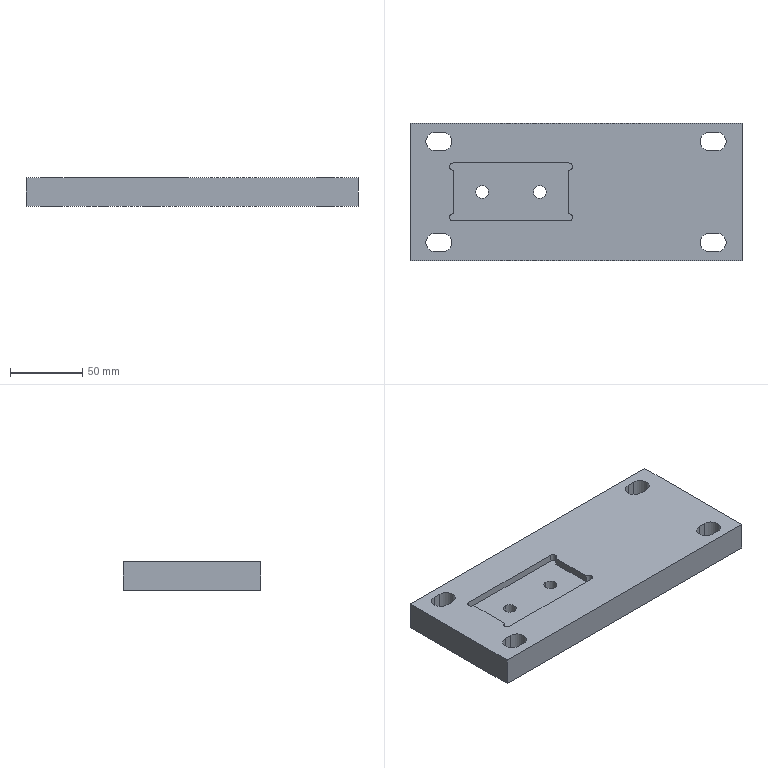CAM job | Mastercam | mm | 12 operations | part box 230 x 95 x 20
1. 2D High Speed (2D Dynamic Mill) | 8 - 8C
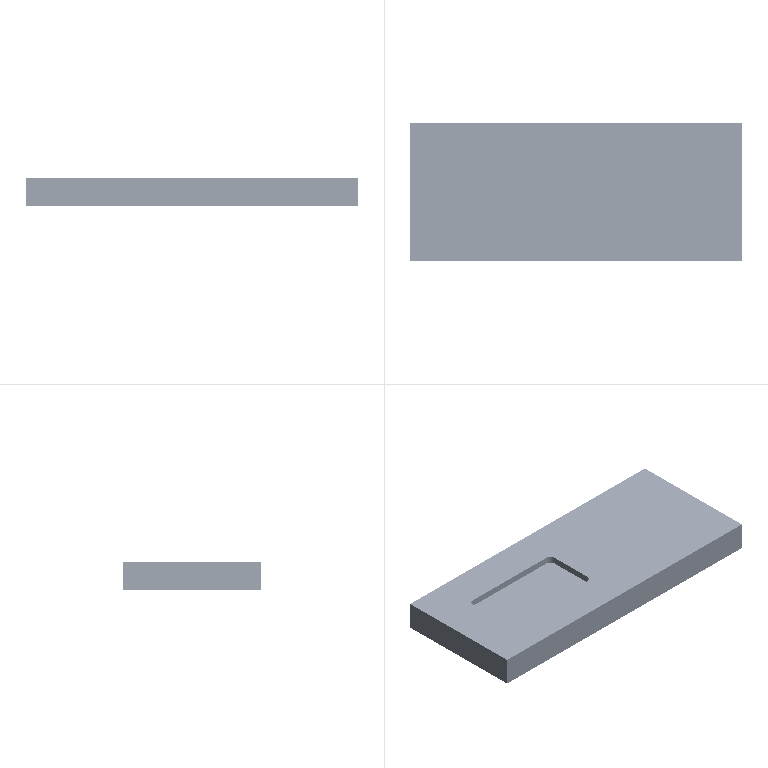2. Contour (Ramp) | 8 - 8C
3. Contour (Ramp) | 8 - 8C
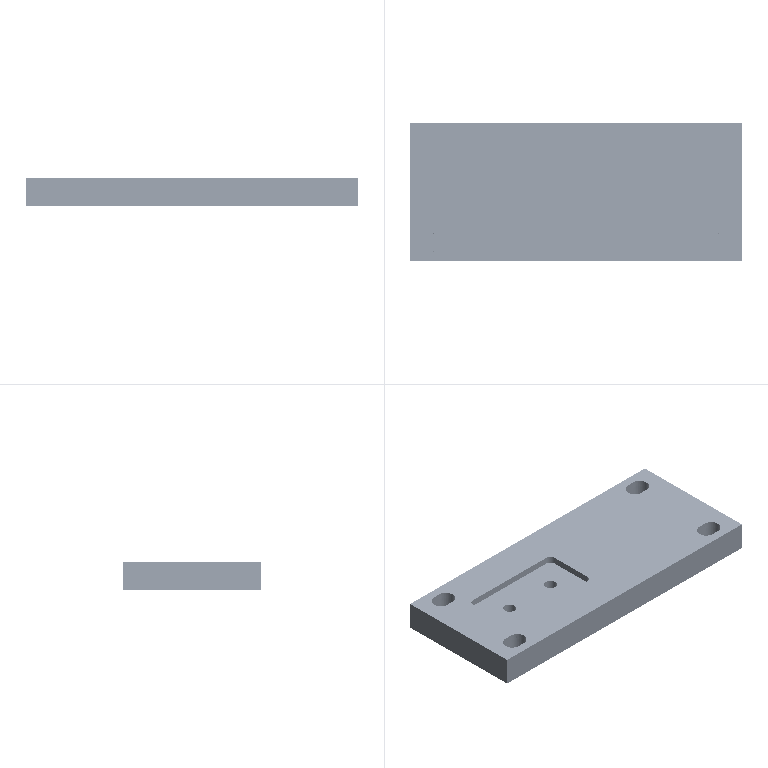4. Pocket (Standard) | 9 - 8J
5. Contour (2D) | 9 - 8J
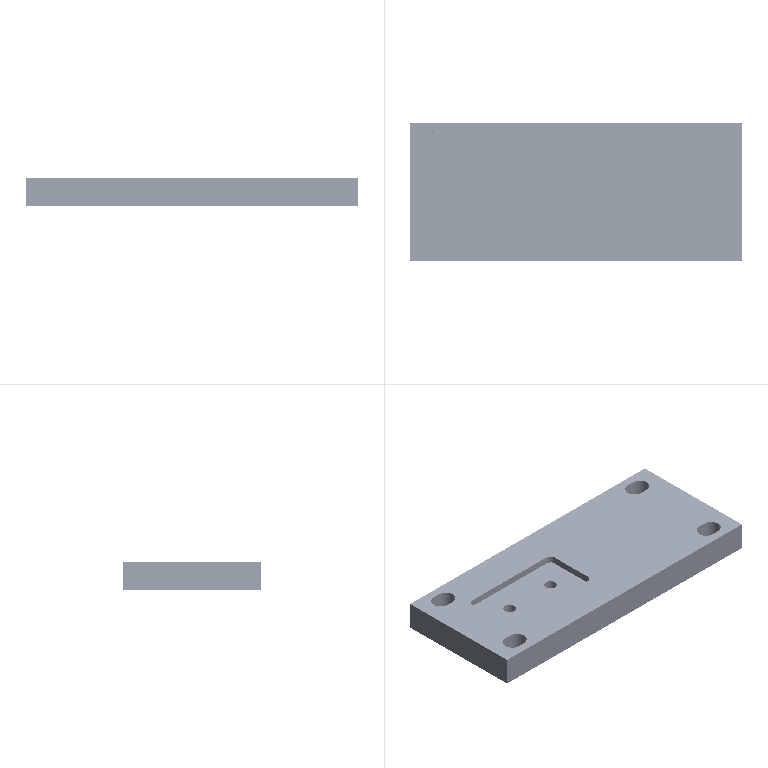6. Contour (2D) | 9 - 8J
7. Contour (Remachining) | 4 - 4C
8. Contour (Remachining) | 5 - 4J
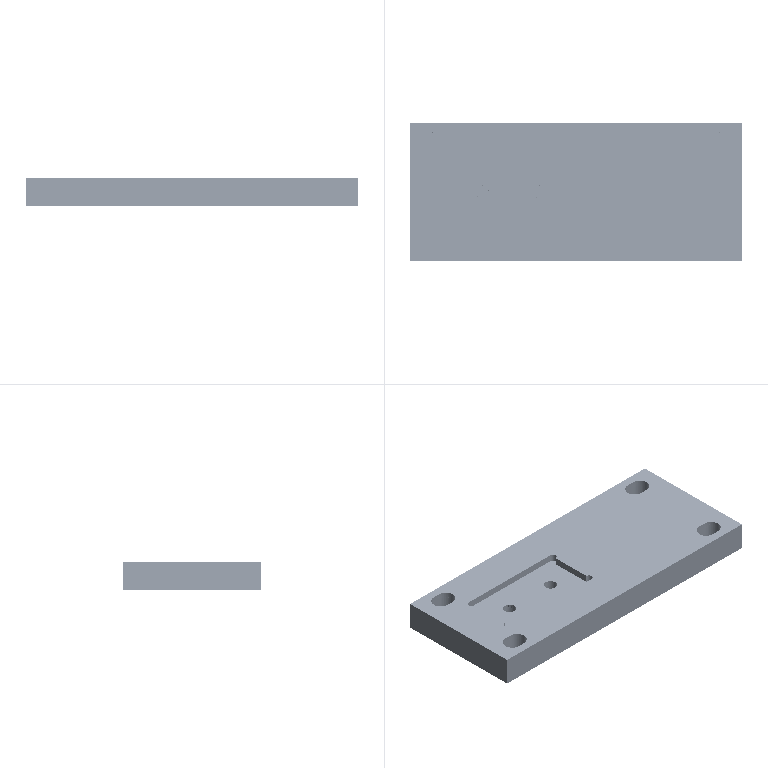9. Model Chamfer | 1 - 6 倒角刀
10. Contour (Ramp) | 8 - 8C
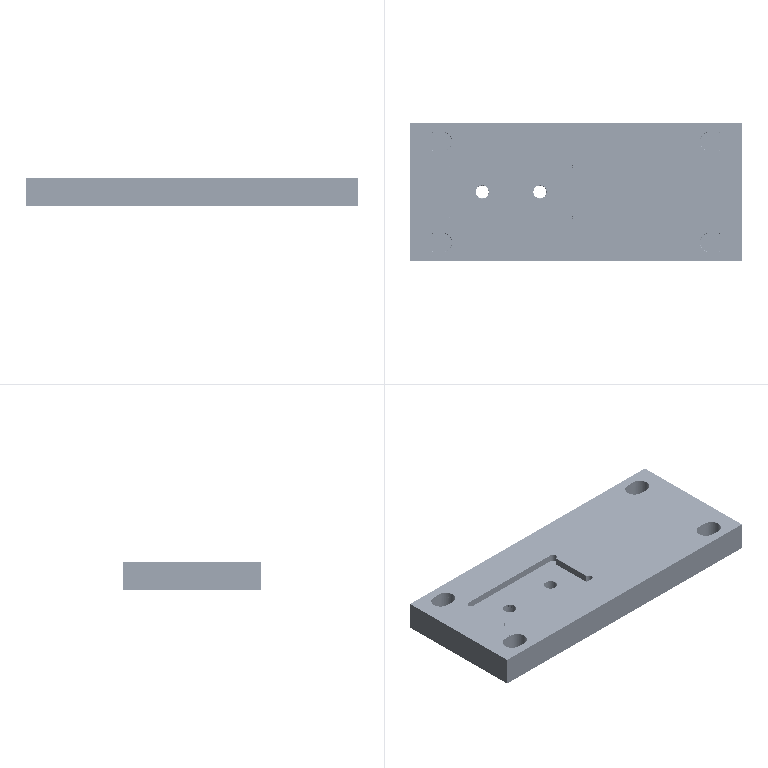11. Contour (2D) | 9 - 8J
12. Model Chamfer | 1 - 6 倒角刀